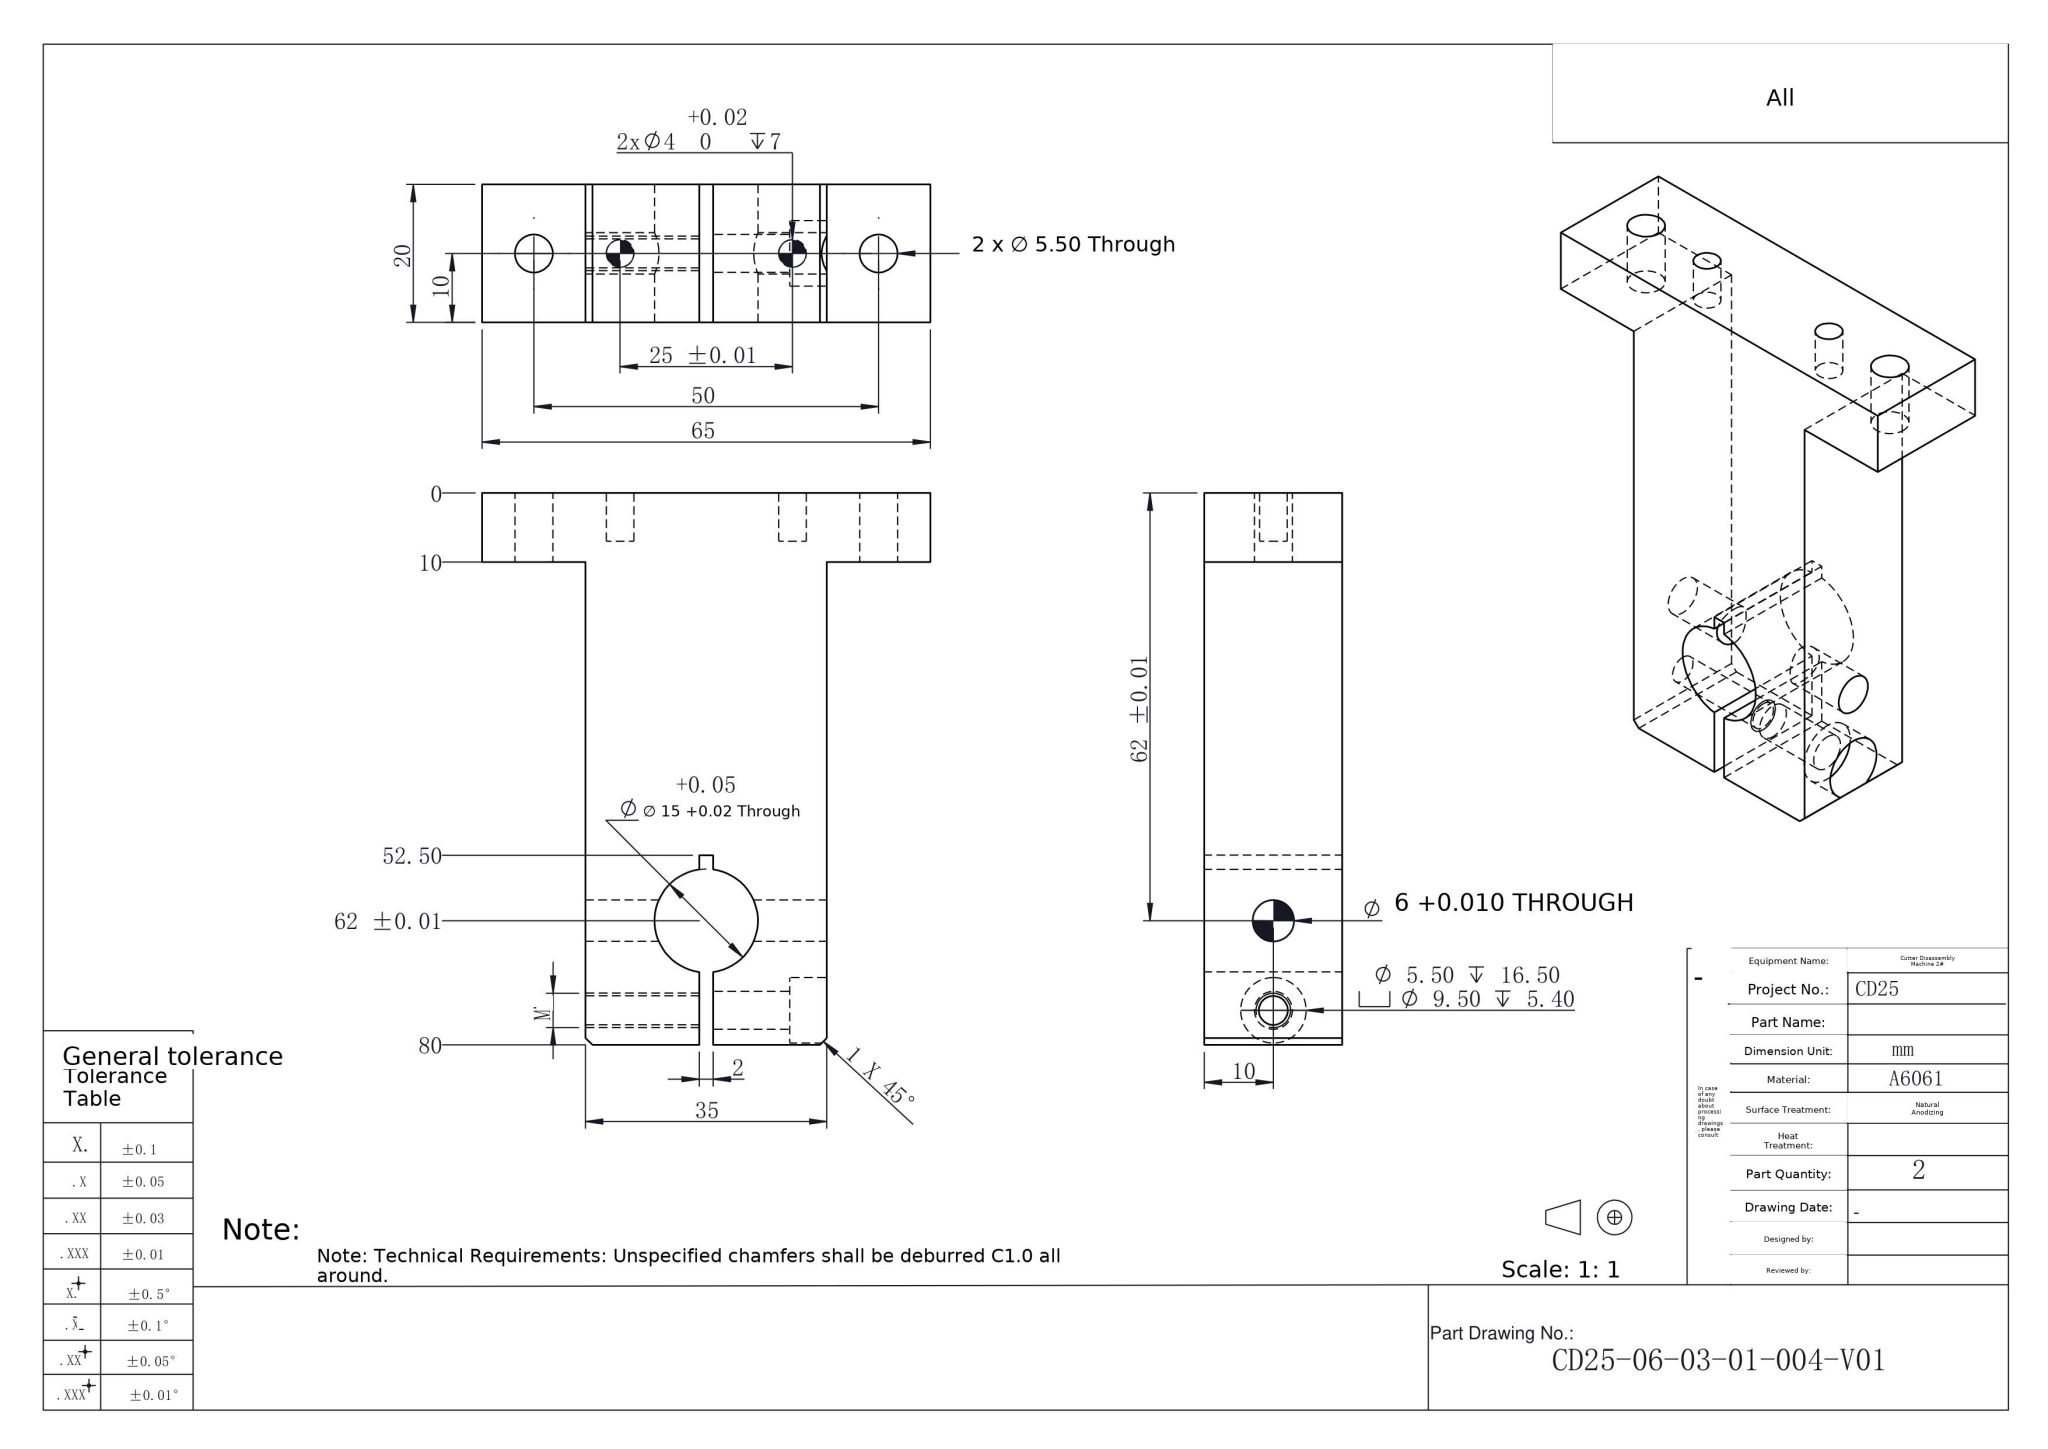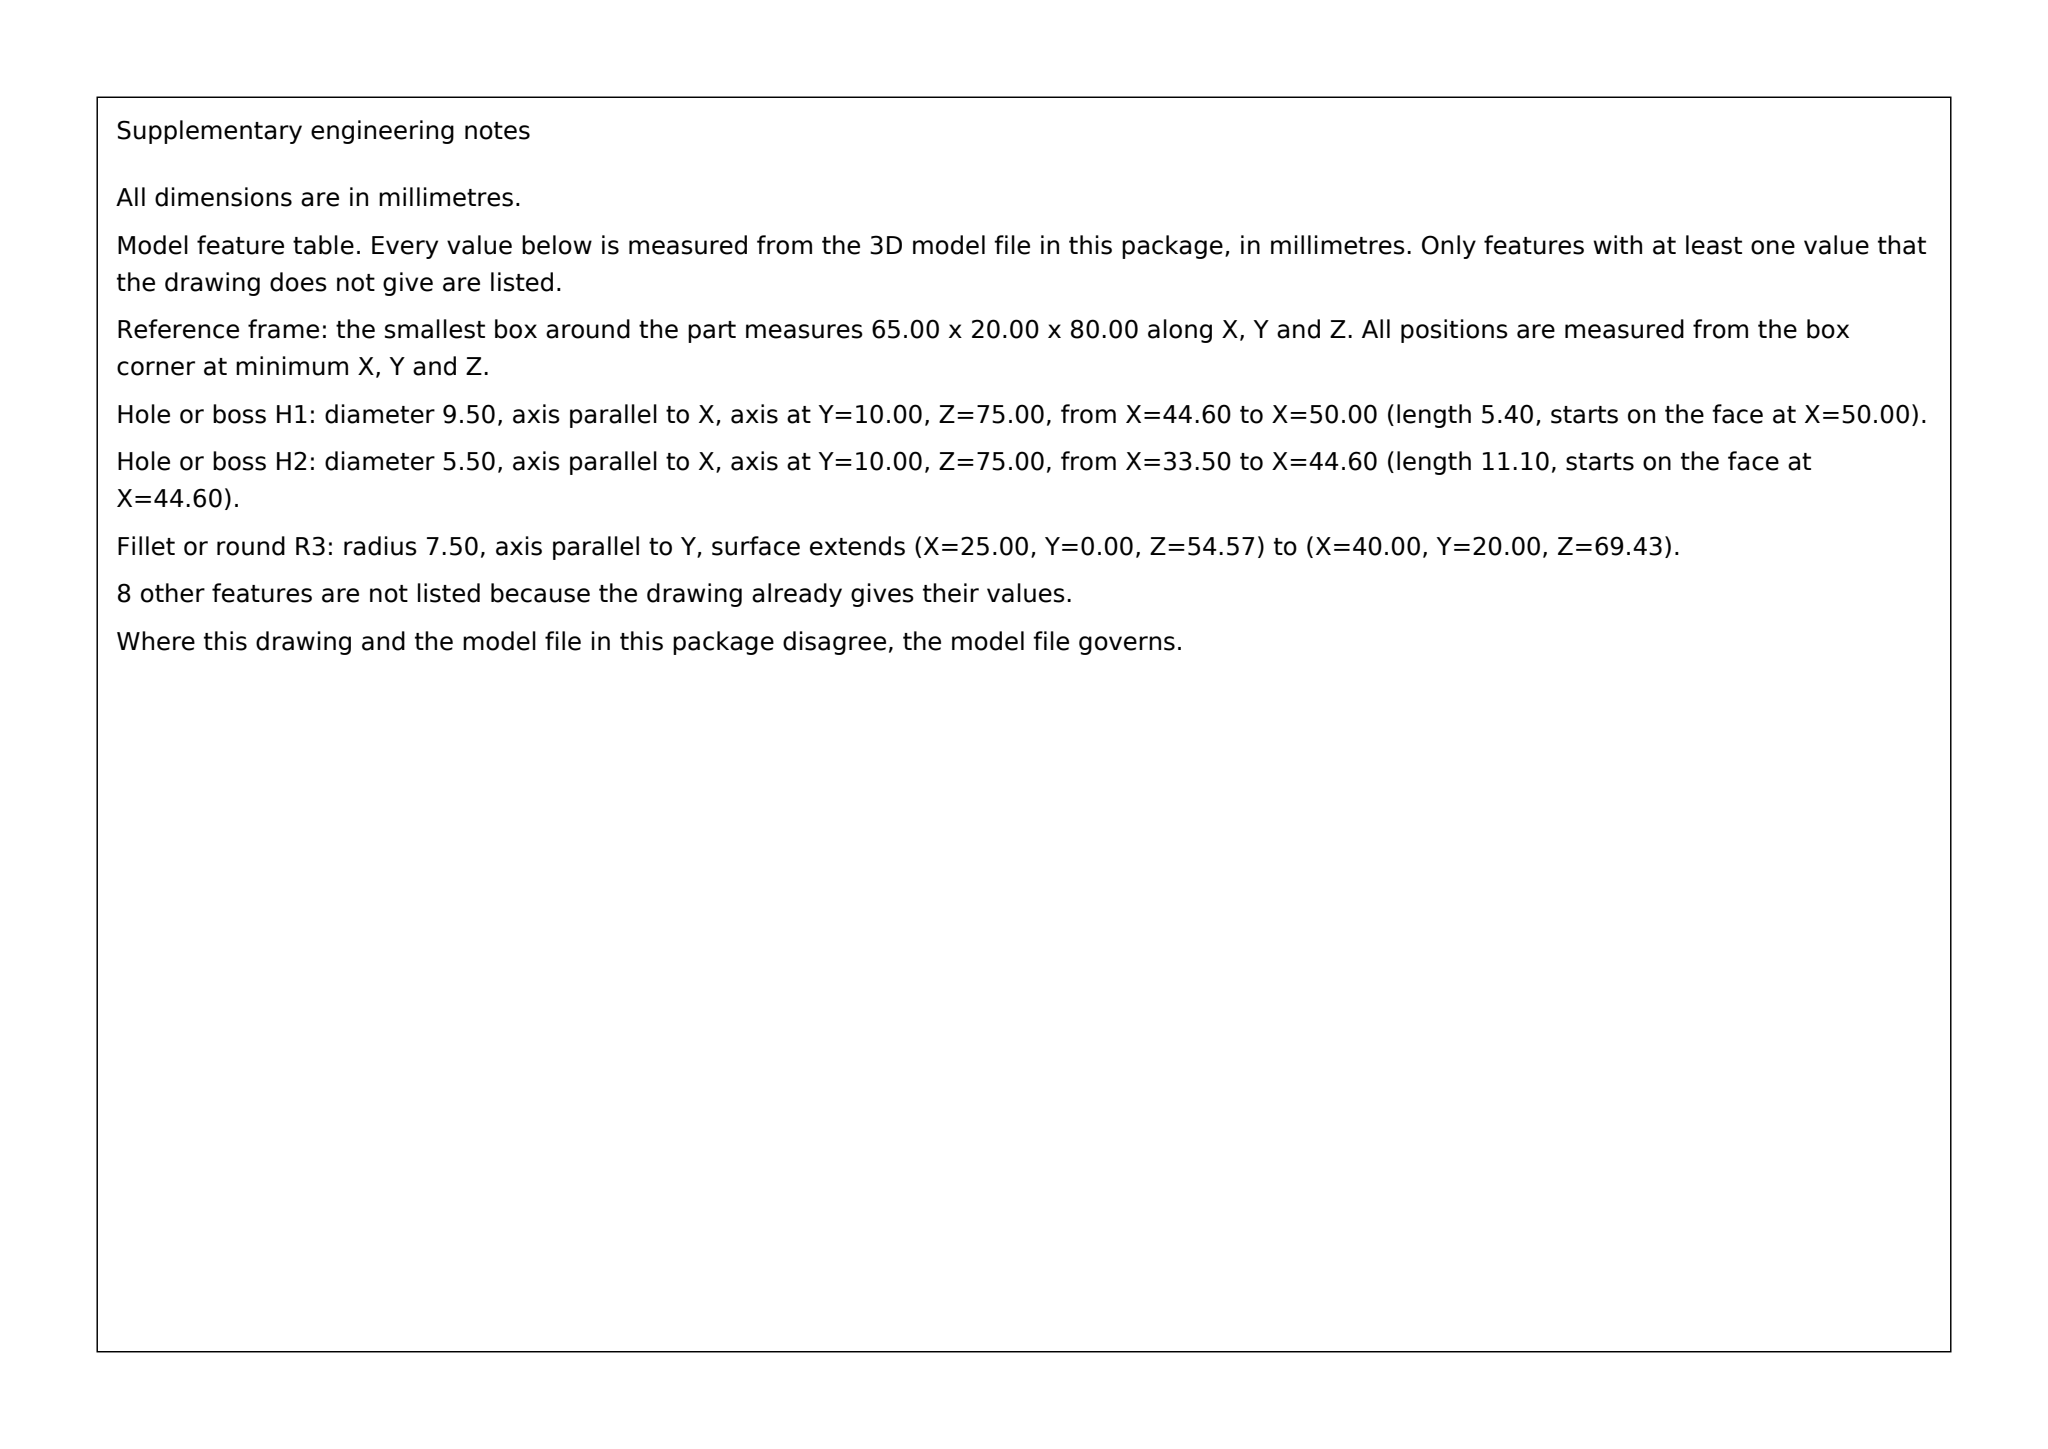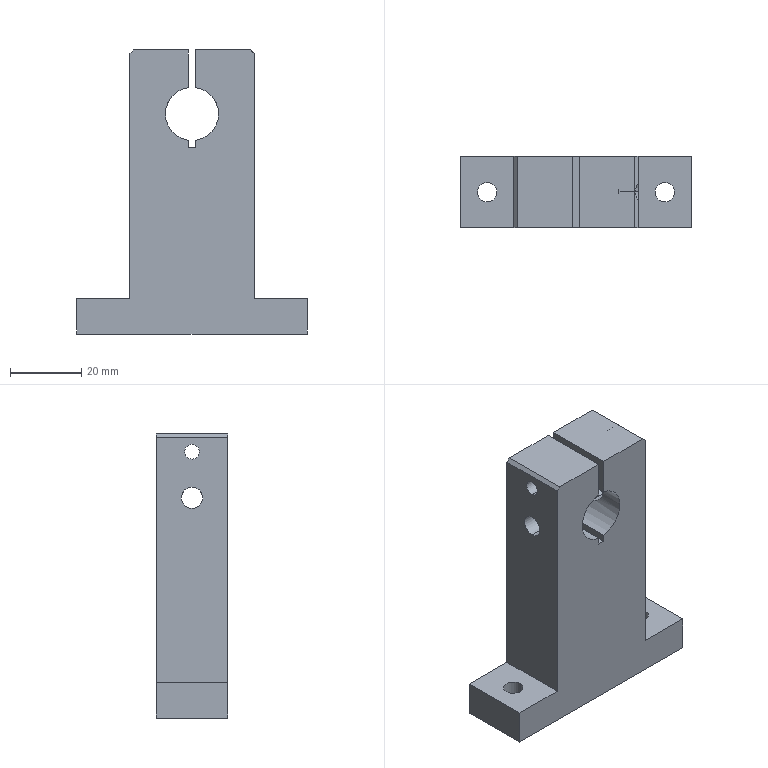Part | SolidWorks | mm | material A6061 | 1 solid | 41 faces | box 65 x 20 x 80 mm | volume 55844 mm3 | plane 21 | cylinder 20 | commonest cylinder face diameters 5.5 x6 4 x4 6 x4 9.5 x2 4.2 x2 15 x2